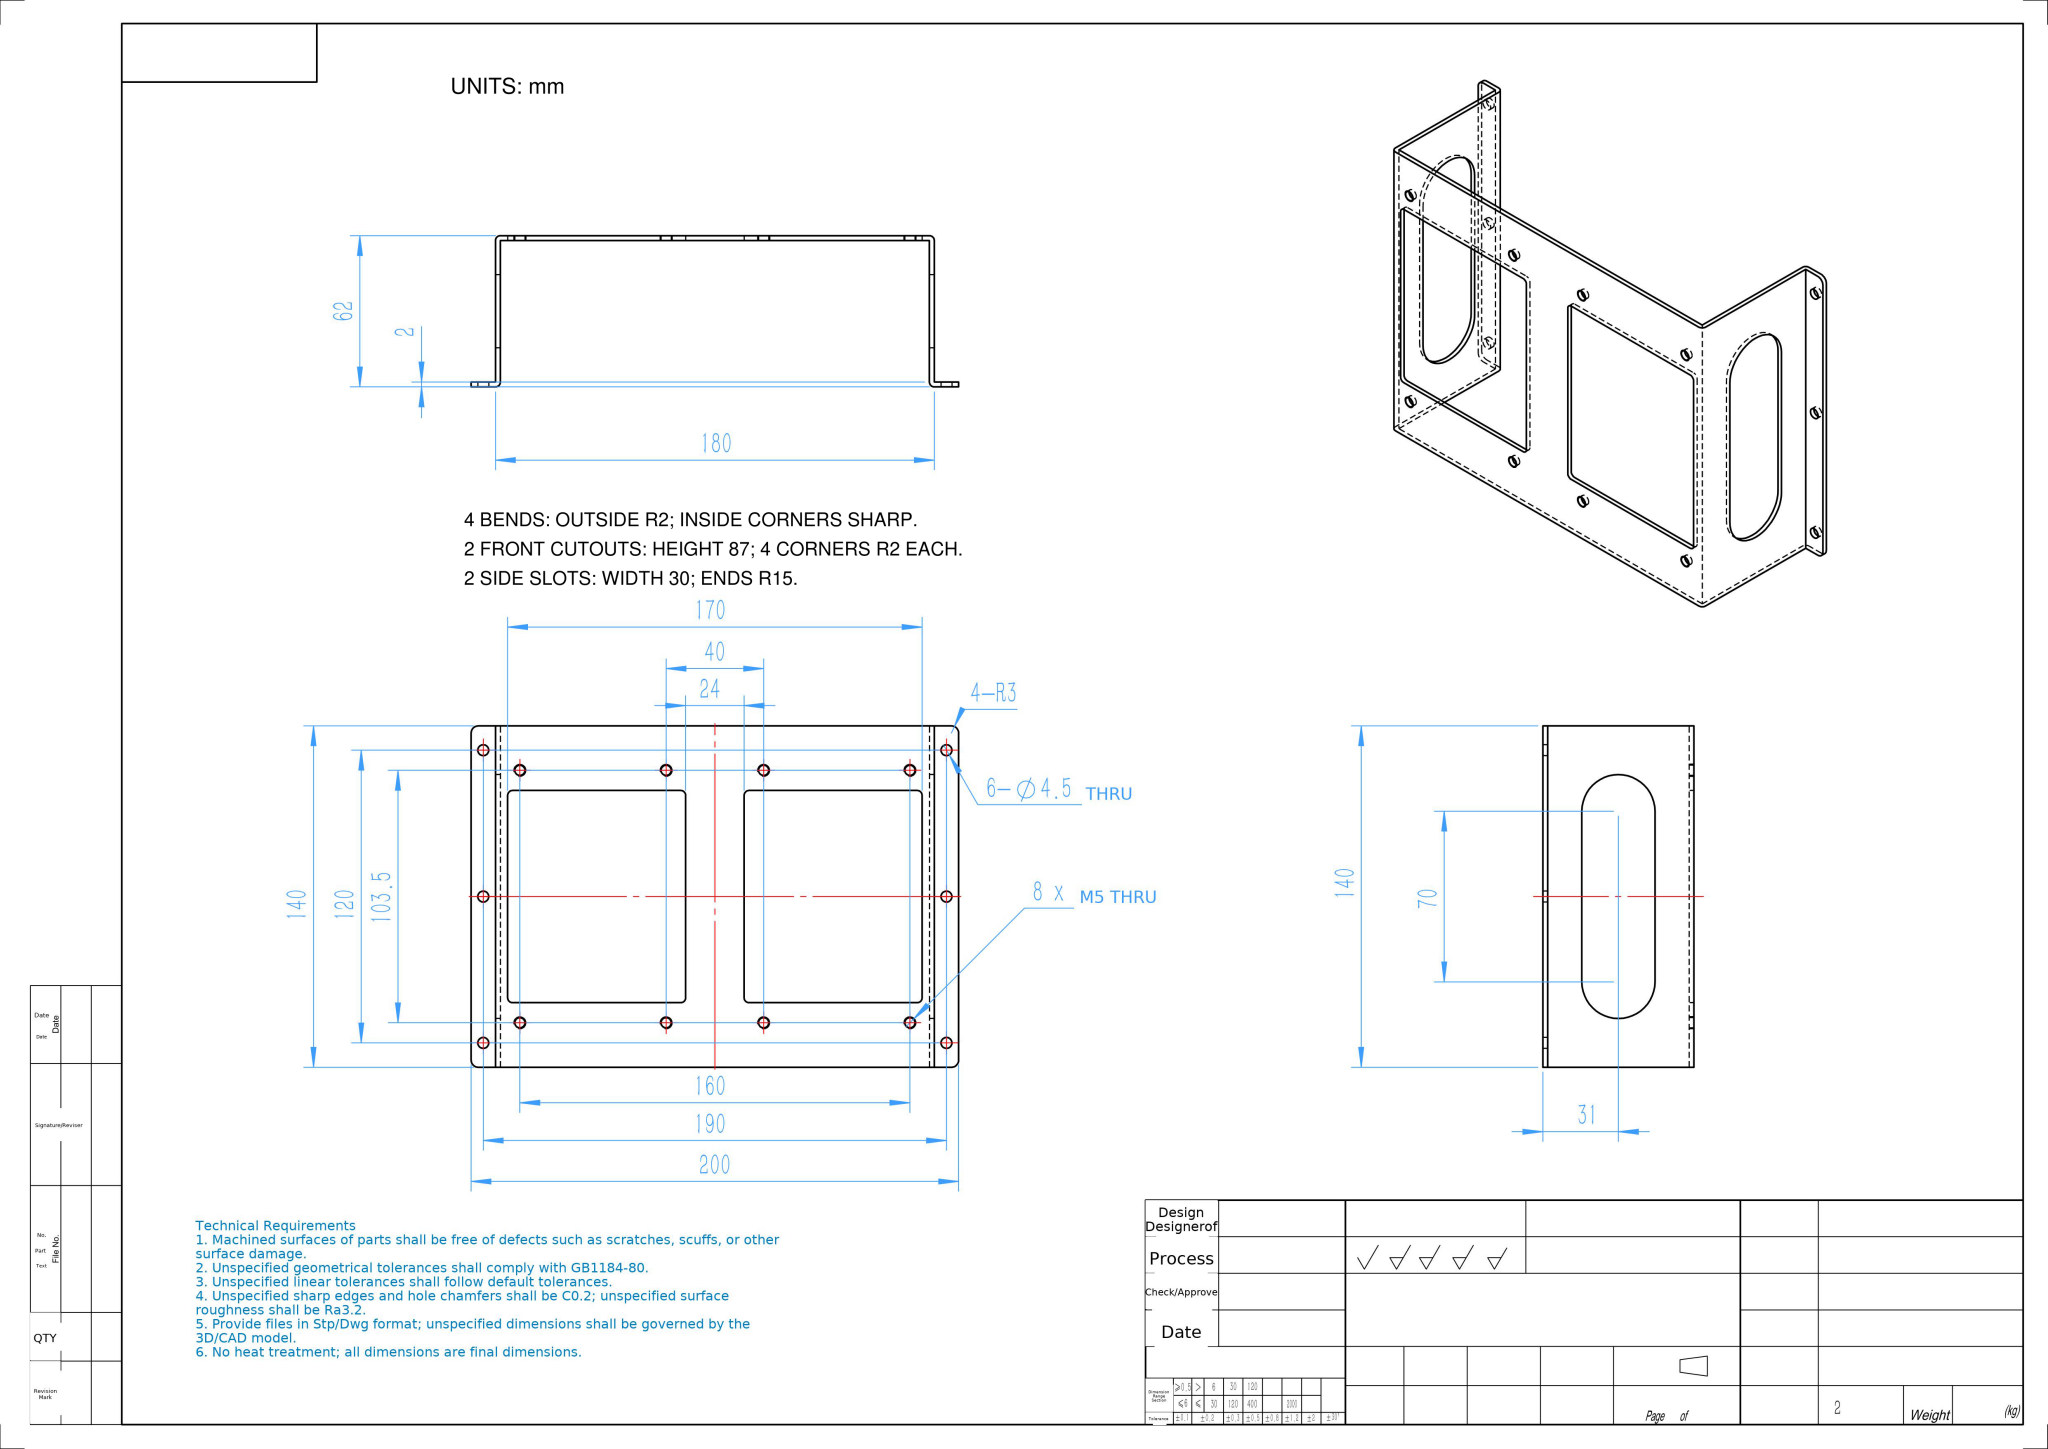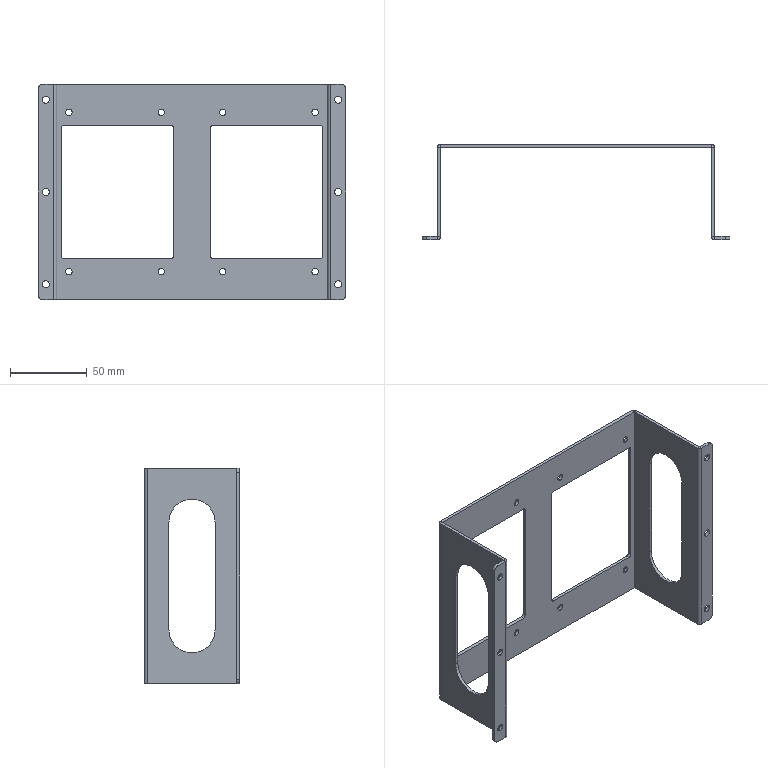Part | NX | mm | 1 solid | 90 faces | box 200 x 62 x 140 mm | volume 52074 mm3 | cylinder 48 | plane 42 | commonest cylinder face diameters 4.2 x16 4.5 x12 4 x12 30 x4 6 x4